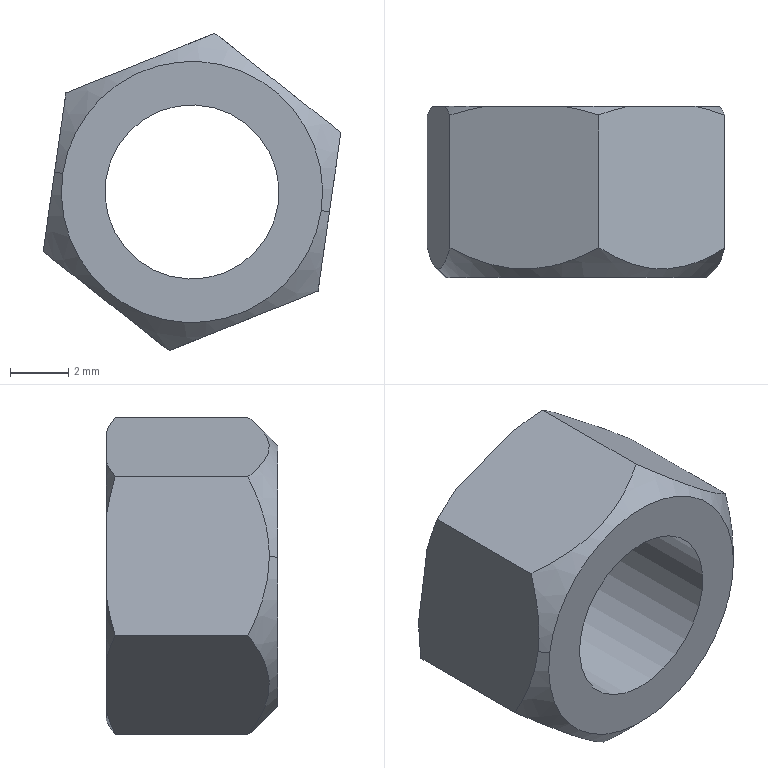Component | NX | HEX_LOCK_NUT_M6_GB_T_6184 | 1 solid | 17 faces | volume 296 mm3 | cone 8 | plane 8 | cylinder 1 | commonest cylinder face diameters 6 x1